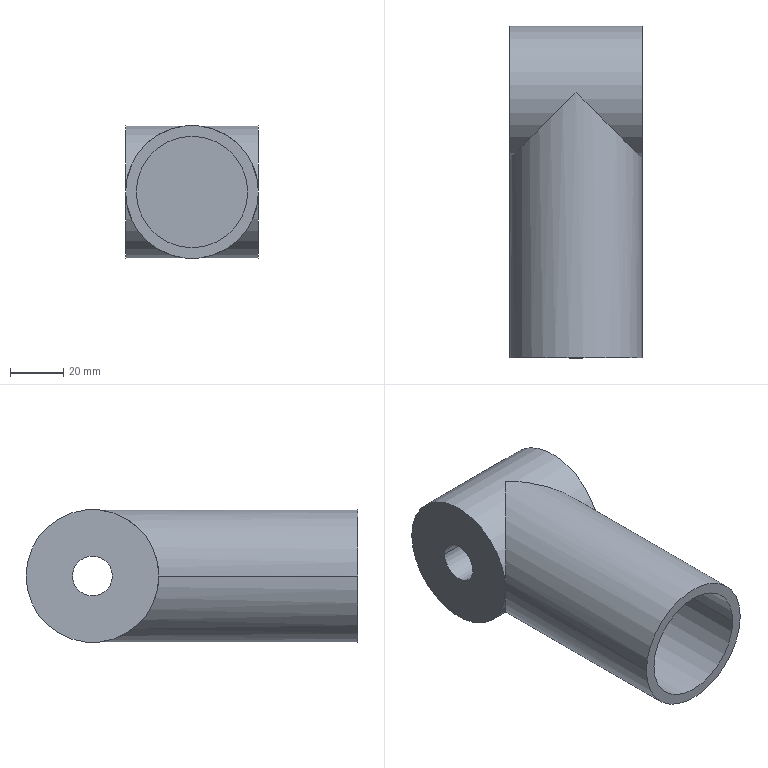Component | SolidWorks | CylinderHousing-2 | 2 solids | 14 faces | box 50 x 125 x 50 mm | volume 147041 mm3 | cylinder 10 | plane 4 | commonest cylinder face diameters 50 x6 42 x2 15 x2
build123d program:
from build123d import *

# Parameters (mm, degrees)
SKETCH1_R                            = 25
SKETCH1_R_2                          = 7.5
BOSS_EXTRUDE1_DEPTH                  = 50
SKETCH3_R                            = 25
BOSS_EXTRUDE2_DEPTH                  = 75
BOSS_EXTRUDE2_DIRECTION_2_REACH      = 334.603
BOSS_EXTRUDE2_DIRECTION_2_END_RADIUS = 25
SKETCH4_R                            = 21
CUT_EXTRUDE1_DEPTH                   = 70


with BuildPart() as part:
    # Sketch1 → Boss-Extrude1 (new body)
    with BuildSketch(Plane.XY):
        with Locations((-135, 300)):
            Circle(SKETCH1_R)
        with Locations((-135, 300)):
            Circle(SKETCH1_R_2, mode=Mode.SUBTRACT)
    extrude(amount=BOSS_EXTRUDE1_DEPTH)


with BuildPart() as body_2:
    # Sketch3 → Boss-Extrude2 (new body)
    with BuildSketch(Plane.ZY.offset(160)):
        with Locations(Location((25, 300, 0), (0, 0, 270))):
            Circle(SKETCH3_R)
    extrude(amount=BOSS_EXTRUDE2_DEPTH)

    # Boss-Extrude2 direction 2: up to this cylinder (the profile starts outside it)
    boss_extrude2_direction_2_end = Plane(origin=(-135, 300, 25), z_dir=(0, 0, -1)) * Cylinder(BOSS_EXTRUDE2_DIRECTION_2_END_RADIUS, 720.206, mode=Mode.PRIVATE)
    # Sketch3 → Boss-Extrude2 direction 2 (add, up to the surface)
    with BuildSketch(Plane.ZY.offset(160), mode=Mode.PRIVATE) as boss_extrude2_direction_2_sk1:
        with Locations(Location((25, 300, 0), (0, 0, 270))):
            Circle(SKETCH3_R)
    boss_extrude2_direction_2_tool1 = extrude(boss_extrude2_direction_2_sk1.sketch, amount=-BOSS_EXTRUDE2_DIRECTION_2_REACH, mode=Mode.PRIVATE) - boss_extrude2_direction_2_end
    add(boss_extrude2_direction_2_tool1.solids().sort_by_distance((-160, 300, 25))[0])
    add(boss_extrude2_direction_2_tool1.solids().sort_by_distance((-160, 300, 25))[1])

    # Sketch4 → Cut-Extrude1 (cut)
    with BuildSketch(Plane.ZY.offset(235)):
        with Locations((25, 300)):
            Circle(SKETCH4_R)
    extrude(amount=-CUT_EXTRUDE1_DEPTH, mode=Mode.SUBTRACT)


solid = Compound([part.part, body_2.part])

# Placed as in the assembly
solid = solid.moved(Location((-250, -100, -600), (90, 90, 0)))
STEP:
#1=COLOUR_RGB('',0.7922,0.8196,0.9333);
#2=FILL_AREA_STYLE_COLOUR('',#1);
#3=FILL_AREA_STYLE('',(#2));
#4=SURFACE_STYLE_FILL_AREA(#3);
#5=SURFACE_SIDE_STYLE('',(#4));
#6=SURFACE_STYLE_USAGE(.BOTH.,#5);
#7=PRESENTATION_STYLE_ASSIGNMENT((#6));
#8=CARTESIAN_POINT('',(-9.843,-9.547,-11.811));
#9=VERTEX_POINT('',#8);
#10=CARTESIAN_POINT('',(-9.843,-8.957,-11.811));
#11=VERTEX_POINT('',#10);
#12=CARTESIAN_POINT('',(-9.843,-9.252,-11.811));
#13=DIRECTION('',(-1.,0.,0.));
#14=DIRECTION('',(0.,1.,0.));
#15=AXIS2_PLACEMENT_3D('',#12,#13,#14);
#16=CIRCLE('',#15,0.2953);
#17=EDGE_CURVE('',#9,#11,#16,.T.);
#18=ORIENTED_EDGE('',*,*,#17,.T.);
#19=CARTESIAN_POINT('',(-7.874,-8.957,-11.811));
#20=VERTEX_POINT('',#19);
#21=CARTESIAN_POINT('',(-9.843,-8.957,-11.811));
#22=DIRECTION('',(1.,-0.,-0.));
#23=VECTOR('',#22,39.37);
#24=LINE('',#21,#23);
#25=EDGE_CURVE('',#11,#20,#24,.T.);
#26=ORIENTED_EDGE('',*,*,#25,.T.);
#27=CARTESIAN_POINT('',(-7.874,-9.547,-11.811));
#28=VERTEX_POINT('',#27);
#29=CARTESIAN_POINT('',(-7.874,-9.252,-11.811));
#30=DIRECTION('',(-1.,0.,0.));
#31=DIRECTION('',(0.,1.,0.));
#32=AXIS2_PLACEMENT_3D('',#29,#30,#31);
#33=CIRCLE('',#32,0.2953);
#34=EDGE_CURVE('',#28,#20,#33,.T.);
#35=ORIENTED_EDGE('',*,*,#34,.F.);
#36=CARTESIAN_POINT('',(-9.843,-9.547,-11.811));
#37=DIRECTION('',(1.,-0.,-0.));
#38=VECTOR('',#37,39.37);
#39=LINE('',#36,#38);
#40=EDGE_CURVE('',#9,#28,#39,.T.);
#41=ORIENTED_EDGE('',*,*,#40,.F.);
#42=EDGE_LOOP('',(#18,#26,#35,#41));
#43=FACE_OUTER_BOUND('',#42,.T.);
#44=CARTESIAN_POINT('',(-9.843,-9.252,-11.811));
#45=DIRECTION('',(1.,-0.,-0.));
#46=DIRECTION('',(0.,-1.,0.));
#47=AXIS2_PLACEMENT_3D('',#44,#45,#46);
#48=CYLINDRICAL_SURFACE('',#47,0.2953);
#49=ADVANCED_FACE('',(#43),#48,.F.);
#50=CARTESIAN_POINT('',(-9.843,-8.268,-11.811));
#51=VERTEX_POINT('',#50);
#52=CARTESIAN_POINT('',(-9.843,-10.236,-11.811));
#53=VERTEX_POINT('',#52);
#54=CARTESIAN_POINT('',(-9.843,-9.252,-11.811));
#55=DIRECTION('',(-1.,0.,0.));
#56=DIRECTION('',(0.,1.,0.));
#57=AXIS2_PLACEMENT_3D('',#54,#55,#56);
#58=CIRCLE('',#57,0.9843);
#59=EDGE_CURVE('',#51,#53,#58,.T.);
#60=ORIENTED_EDGE('',*,*,#59,.F.);
#61=CARTESIAN_POINT('',(-7.874,-8.268,-11.811));
#62=VERTEX_POINT('',#61);
#63=CARTESIAN_POINT('',(-9.843,-8.268,-11.811));
#64=DIRECTION('',(1.,-0.,-0.));
#65=VECTOR('',#64,39.37);
#66=LINE('',#63,#65);
#67=EDGE_CURVE('',#51,#62,#66,.T.);
#68=ORIENTED_EDGE('',*,*,#67,.T.);
#69=CARTESIAN_POINT('',(-7.874,-10.236,-11.811));
#70=VERTEX_POINT('',#69);
#71=CARTESIAN_POINT('',(-7.874,-9.252,-11.811));
#72=DIRECTION('',(-1.,0.,0.));
#73=DIRECTION('',(0.,1.,0.));
#74=AXIS2_PLACEMENT_3D('',#71,#72,#73);
#75=CIRCLE('',#74,0.9843);
#76=EDGE_CURVE('',#62,#70,#75,.T.);
#77=ORIENTED_EDGE('',*,*,#76,.T.);
#78=CARTESIAN_POINT('',(-9.843,-10.236,-11.811));
#79=DIRECTION('',(1.,-0.,-0.));
#80=VECTOR('',#79,39.37);
#81=LINE('',#78,#80);
#82=EDGE_CURVE('',#53,#70,#81,.T.);
#83=ORIENTED_EDGE('',*,*,#82,.F.);
#84=EDGE_LOOP('',(#60,#68,#77,#83));
#85=FACE_OUTER_BOUND('',#84,.T.);
#86=CARTESIAN_POINT('',(-9.843,-9.252,-11.811));
#87=DIRECTION('',(1.,-0.,-0.));
#88=DIRECTION('',(0.,-1.,0.));
#89=AXIS2_PLACEMENT_3D('',#86,#87,#88);
#90=CYLINDRICAL_SURFACE('',#89,0.9843);
#91=ADVANCED_FACE('',(#85),#90,.T.);
#92=CARTESIAN_POINT('',(-9.843,-9.252,-11.811));
#93=DIRECTION('',(-1.,0.,0.));
#94=DIRECTION('',(0.,1.,0.));
#95=AXIS2_PLACEMENT_3D('',#92,#93,#94);
#96=CIRCLE('',#95,0.9843);
#97=EDGE_CURVE('',#53,#51,#96,.T.);
#98=ORIENTED_EDGE('',*,*,#97,.T.);
#99=ORIENTED_EDGE('',*,*,#59,.T.);
#100=EDGE_LOOP('',(#98,#99));
#101=FACE_OUTER_BOUND('',#100,.T.);
#102=ORIENTED_EDGE('',*,*,#17,.F.);
#103=CARTESIAN_POINT('',(-9.843,-9.252,-11.811));
#104=DIRECTION('',(-1.,0.,0.));
#105=DIRECTION('',(0.,1.,0.));
#106=AXIS2_PLACEMENT_3D('',#103,#104,#105);
#107=CIRCLE('',#106,0.2953);
#108=EDGE_CURVE('',#11,#9,#107,.T.);
#109=ORIENTED_EDGE('',*,*,#108,.F.);
#110=EDGE_LOOP('',(#102,#109));
#111=FACE_BOUND('',#110,.T.);
#112=CARTESIAN_POINT('',(-9.843,-9.252,-11.811));
#113=DIRECTION('',(-1.,0.,0.));
#114=DIRECTION('',(0.,1.,0.));
#115=AXIS2_PLACEMENT_3D('',#112,#113,#114);
#116=PLANE('',#115);
#117=ADVANCED_FACE('',(#101,#111),#116,.T.);
#118=CARTESIAN_POINT('',(-7.874,-9.252,-11.811));
#119=DIRECTION('',(-1.,0.,0.));
#120=DIRECTION('',(0.,1.,0.));
#121=AXIS2_PLACEMENT_3D('',#118,#119,#120);
#122=CIRCLE('',#121,0.9843);
#123=EDGE_CURVE('',#70,#62,#122,.T.);
#124=ORIENTED_EDGE('',*,*,#123,.F.);
#125=ORIENTED_EDGE('',*,*,#76,.F.);
#126=EDGE_LOOP('',(#124,#125));
#127=FACE_OUTER_BOUND('',#126,.T.);
#128=ORIENTED_EDGE('',*,*,#34,.T.);
#129=CARTESIAN_POINT('',(-7.874,-9.252,-11.811));
#130=DIRECTION('',(-1.,0.,0.));
#131=DIRECTION('',(0.,1.,0.));
#132=AXIS2_PLACEMENT_3D('',#129,#130,#131);
#133=CIRCLE('',#132,0.2953);
#134=EDGE_CURVE('',#20,#28,#133,.T.);
#135=ORIENTED_EDGE('',*,*,#134,.T.);
#136=EDGE_LOOP('',(#128,#135));
#137=FACE_BOUND('',#136,.T.);
#138=CARTESIAN_POINT('',(-7.874,-9.252,-11.811));
#139=DIRECTION('',(-1.,0.,0.));
#140=DIRECTION('',(0.,1.,0.));
#141=AXIS2_PLACEMENT_3D('',#138,#139,#140);
#142=PLANE('',#141);
#143=ADVANCED_FACE('',(#127,#137),#142,.F.);
#144=ORIENTED_EDGE('',*,*,#67,.F.);
#145=ORIENTED_EDGE('',*,*,#97,.F.);
#146=ORIENTED_EDGE('',*,*,#82,.T.);
#147=ORIENTED_EDGE('',*,*,#123,.T.);
#148=EDGE_LOOP('',(#144,#145,#146,#147));
#149=FACE_OUTER_BOUND('',#148,.T.);
#150=CARTESIAN_POINT('',(-9.843,-9.252,-11.811));
#151=DIRECTION('',(1.,-0.,-0.));
#152=DIRECTION('',(0.,-1.,0.));
#153=AXIS2_PLACEMENT_3D('',#150,#151,#152);
#154=CYLINDRICAL_SURFACE('',#153,0.9843);
#155=ADVANCED_FACE('',(#149),#154,.T.);
#156=ORIENTED_EDGE('',*,*,#25,.F.);
#157=ORIENTED_EDGE('',*,*,#108,.T.);
#158=ORIENTED_EDGE('',*,*,#40,.T.);
#159=ORIENTED_EDGE('',*,*,#134,.F.);
#160=EDGE_LOOP('',(#156,#157,#158,#159));
#161=FACE_OUTER_BOUND('',#160,.T.);
#162=CARTESIAN_POINT('',(-9.843,-9.252,-11.811));
#163=DIRECTION('',(1.,-0.,-0.));
#164=DIRECTION('',(0.,-1.,0.));
#165=AXIS2_PLACEMENT_3D('',#162,#163,#164);
#166=CYLINDRICAL_SURFACE('',#165,0.2953);
#167=ADVANCED_FACE('',(#161),#166,.F.);
#168=CLOSED_SHELL('',(#49,#91,#117,#143,#155,#167));
#169=MANIFOLD_SOLID_BREP('',#168);
#170=STYLED_ITEM('',(#7),#169);
#171=PRESENTATION_LAYER_ASSIGNMENT('','',(#170));
#172=COLOUR_RGB('',0.7922,0.8196,0.9333);
#173=FILL_AREA_STYLE_COLOUR('',#172);
#174=FILL_AREA_STYLE('',(#173));
#175=SURFACE_STYLE_FILL_AREA(#174);
#176=SURFACE_SIDE_STYLE('',(#175));
#177=SURFACE_STYLE_USAGE(.BOTH.,#176);
#178=PRESENTATION_STYLE_ASSIGNMENT((#177));
#179=CARTESIAN_POINT('',(-8.031,-10.433,-11.811));
#180=VERTEX_POINT('',#179);
#181=CARTESIAN_POINT('',(-9.685,-10.433,-11.811));
#182=VERTEX_POINT('',#181);
#183=CARTESIAN_POINT('',(-8.858,-10.433,-11.811));
#184=DIRECTION('',(-0.,-1.,-0.));
#185=DIRECTION('',(-1.,0.,0.));
#186=AXIS2_PLACEMENT_3D('',#183,#184,#185);
#187=CIRCLE('',#186,0.8268);
#188=EDGE_CURVE('',#180,#182,#187,.T.);
#189=ORIENTED_EDGE('',*,*,#188,.F.);
#190=CARTESIAN_POINT('',(-8.031,-13.189,-11.811));
#191=VERTEX_POINT('',#190);
#192=CARTESIAN_POINT('',(-8.031,-10.433,-11.811));
#193=DIRECTION('',(-0.,-1.,-0.));
#194=VECTOR('',#193,39.37);
#195=LINE('',#192,#194);
#196=EDGE_CURVE('',#180,#191,#195,.T.);
#197=ORIENTED_EDGE('',*,*,#196,.T.);
#198=CARTESIAN_POINT('',(-9.685,-13.189,-11.811));
#199=VERTEX_POINT('',#198);
#200=CARTESIAN_POINT('',(-8.858,-13.189,-11.811));
#201=DIRECTION('',(-0.,-1.,-0.));
#202=DIRECTION('',(-1.,0.,0.));
#203=AXIS2_PLACEMENT_3D('',#200,#201,#202);
#204=CIRCLE('',#203,0.8268);
#205=EDGE_CURVE('',#191,#199,#204,.T.);
#206=ORIENTED_EDGE('',*,*,#205,.T.);
#207=CARTESIAN_POINT('',(-9.685,-10.433,-11.811));
#208=DIRECTION('',(-0.,-1.,-0.));
#209=VECTOR('',#208,39.37);
#210=LINE('',#207,#209);
#211=EDGE_CURVE('',#182,#199,#210,.T.);
#212=ORIENTED_EDGE('',*,*,#211,.F.);
#213=EDGE_LOOP('',(#189,#197,#206,#212));
#214=FACE_OUTER_BOUND('',#213,.T.);
#215=CARTESIAN_POINT('',(-8.858,-10.433,-11.811));
#216=DIRECTION('',(-0.,-1.,-0.));
#217=DIRECTION('',(-1.,0.,0.));
#218=AXIS2_PLACEMENT_3D('',#215,#216,#217);
#219=CYLINDRICAL_SURFACE('',#218,0.8268);
#220=ADVANCED_FACE('',(#214),#219,.F.);
#221=CARTESIAN_POINT('',(-9.843,-10.236,-11.811));
#222=VERTEX_POINT('',#221);
#223=CARTESIAN_POINT('',(-8.858,-9.252,-12.795));
#224=VERTEX_POINT('',#223);
#225=CARTESIAN_POINT('',(-9.843,-10.236,-11.811));
#226=CARTESIAN_POINT('',(-9.843,-10.236,-12.388));
#227=CARTESIAN_POINT('',(-9.435,-9.829,-12.795));
#228=CARTESIAN_POINT('',(-8.858,-9.252,-12.795));
#229=(BOUNDED_CURVE()B_SPLINE_CURVE(3,(#225,#226,#227,#228),.UNSPECIFIED.,.F.,.T.)B_SPLINE_CURVE_WITH_KNOTS((4,4),(-0.,1.571),.UNSPECIFIED.)CURVE()GEOMETRIC_REPRESENTATION_ITEM()RATIONAL_B_SPLINE_CURVE((1.,0.8047,0.8047,1.))REPRESENTATION_ITEM(''));
#230=EDGE_CURVE('',#222,#224,#229,.T.);
#231=ORIENTED_EDGE('',*,*,#230,.F.);
#232=CARTESIAN_POINT('',(-7.874,-10.236,-11.811));
#233=VERTEX_POINT('',#232);
#234=CARTESIAN_POINT('',(-9.843,-10.236,-11.811));
#235=DIRECTION('',(1.,-0.,-0.));
#236=VECTOR('',#235,39.37);
#237=LINE('',#234,#236);
#238=EDGE_CURVE('',#222,#233,#237,.T.);
#239=ORIENTED_EDGE('',*,*,#238,.T.);
#240=CARTESIAN_POINT('',(-8.858,-9.252,-12.795));
#241=CARTESIAN_POINT('',(-8.282,-9.829,-12.795));
#242=CARTESIAN_POINT('',(-7.874,-10.236,-12.388));
#243=CARTESIAN_POINT('',(-7.874,-10.236,-11.811));
#244=(BOUNDED_CURVE()B_SPLINE_CURVE(3,(#240,#241,#242,#243),.UNSPECIFIED.,.F.,.F.)B_SPLINE_CURVE_WITH_KNOTS((4,4),(4.712,6.283),.UNSPECIFIED.)CURVE()GEOMETRIC_REPRESENTATION_ITEM()RATIONAL_B_SPLINE_CURVE((1.,0.8047,0.8047,1.))REPRESENTATION_ITEM(''));
#245=EDGE_CURVE('',#224,#233,#244,.T.);
#246=ORIENTED_EDGE('',*,*,#245,.F.);
#247=EDGE_LOOP('',(#231,#239,#246));
#248=FACE_OUTER_BOUND('',#247,.T.);
#249=CARTESIAN_POINT('',(-9.843,-9.252,-11.811));
#250=DIRECTION('',(1.,-0.,-0.));
#251=DIRECTION('',(0.,-1.,0.));
#252=AXIS2_PLACEMENT_3D('',#249,#250,#251);
#253=CYLINDRICAL_SURFACE('',#252,0.9843);
#254=ADVANCED_FACE('',(#248),#253,.F.);
#255=CARTESIAN_POINT('',(-9.843,-13.189,-11.811));
#256=VERTEX_POINT('',#255);
#257=CARTESIAN_POINT('',(-7.874,-13.189,-11.811));
#258=VERTEX_POINT('',#257);
#259=CARTESIAN_POINT('',(-8.858,-13.189,-11.811));
#260=DIRECTION('',(-0.,-1.,-0.));
#261=DIRECTION('',(-1.,0.,0.));
#262=AXIS2_PLACEMENT_3D('',#259,#260,#261);
#263=CIRCLE('',#262,0.9843);
#264=EDGE_CURVE('',#256,#258,#263,.T.);
#265=ORIENTED_EDGE('',*,*,#264,.F.);
#266=CARTESIAN_POINT('',(-9.843,-13.189,-11.811));
#267=DIRECTION('',(0.,1.,0.));
#268=VECTOR('',#267,39.37);
#269=LINE('',#266,#268);
#270=EDGE_CURVE('',#256,#222,#269,.T.);
#271=ORIENTED_EDGE('',*,*,#270,.T.);
#272=ORIENTED_EDGE('',*,*,#230,.T.);
#273=ORIENTED_EDGE('',*,*,#245,.T.);
#274=CARTESIAN_POINT('',(-7.874,-13.189,-11.811));
#275=DIRECTION('',(0.,1.,0.));
#276=VECTOR('',#275,39.37);
#277=LINE('',#274,#276);
#278=EDGE_CURVE('',#258,#233,#277,.T.);
#279=ORIENTED_EDGE('',*,*,#278,.F.);
#280=EDGE_LOOP('',(#265,#271,#272,#273,#279));
#281=FACE_OUTER_BOUND('',#280,.T.);
#282=CARTESIAN_POINT('',(-8.858,-13.189,-11.811));
#283=DIRECTION('',(0.,1.,0.));
#284=DIRECTION('',(1.,0.,0.));
#285=AXIS2_PLACEMENT_3D('',#282,#283,#284);
#286=CYLINDRICAL_SURFACE('',#285,0.9843);
#287=ADVANCED_FACE('',(#281),#286,.T.);
#288=ORIENTED_EDGE('',*,*,#270,.F.);
#289=CARTESIAN_POINT('',(-8.858,-13.189,-11.811));
#290=DIRECTION('',(-0.,-1.,-0.));
#291=DIRECTION('',(-1.,0.,0.));
#292=AXIS2_PLACEMENT_3D('',#289,#290,#291);
#293=CIRCLE('',#292,0.9843);
#294=EDGE_CURVE('',#258,#256,#293,.T.);
#295=ORIENTED_EDGE('',*,*,#294,.F.);
#296=ORIENTED_EDGE('',*,*,#278,.T.);
#297=CARTESIAN_POINT('',(-8.858,-9.252,-10.827));
#298=VERTEX_POINT('',#297);
#299=CARTESIAN_POINT('',(-7.874,-10.236,-11.811));
#300=CARTESIAN_POINT('',(-7.874,-10.236,-11.234));
#301=CARTESIAN_POINT('',(-8.282,-9.829,-10.827));
#302=CARTESIAN_POINT('',(-8.858,-9.252,-10.827));
#303=(BOUNDED_CURVE()B_SPLINE_CURVE(3,(#299,#300,#301,#302),.UNSPECIFIED.,.F.,.T.)B_SPLINE_CURVE_WITH_KNOTS((4,4),(0.,1.571),.UNSPECIFIED.)CURVE()GEOMETRIC_REPRESENTATION_ITEM()RATIONAL_B_SPLINE_CURVE((1.,0.8047,0.8047,1.))REPRESENTATION_ITEM(''));
#304=EDGE_CURVE('',#233,#298,#303,.T.);
#305=ORIENTED_EDGE('',*,*,#304,.T.);
#306=CARTESIAN_POINT('',(-8.858,-9.252,-10.827));
#307=CARTESIAN_POINT('',(-9.435,-9.829,-10.827));
#308=CARTESIAN_POINT('',(-9.843,-10.236,-11.234));
#309=CARTESIAN_POINT('',(-9.843,-10.236,-11.811));
#310=(BOUNDED_CURVE()B_SPLINE_CURVE(3,(#306,#307,#308,#309),.UNSPECIFIED.,.F.,.T.)B_SPLINE_CURVE_WITH_KNOTS((4,4),(4.712,6.283),.UNSPECIFIED.)CURVE()GEOMETRIC_REPRESENTATION_ITEM()RATIONAL_B_SPLINE_CURVE((1.,0.8047,0.8047,1.))REPRESENTATION_ITEM(''));
#311=EDGE_CURVE('',#298,#222,#310,.T.);
#312=ORIENTED_EDGE('',*,*,#311,.T.);
#313=EDGE_LOOP('',(#288,#295,#296,#305,#312));
#314=FACE_OUTER_BOUND('',#313,.T.);
#315=CARTESIAN_POINT('',(-8.858,-13.189,-11.811));
#316=DIRECTION('',(0.,1.,0.));
#317=DIRECTION('',(1.,0.,0.));
#318=AXIS2_PLACEMENT_3D('',#315,#316,#317);
#319=CYLINDRICAL_SURFACE('',#318,0.9843);
#320=ADVANCED_FACE('',(#314),#319,.T.);
#321=CARTESIAN_POINT('',(-8.858,-13.189,-11.811));
#322=DIRECTION('',(-0.,-1.,-0.));
#323=DIRECTION('',(-1.,0.,0.));
#324=AXIS2_PLACEMENT_3D('',#321,#322,#323);
#325=CIRCLE('',#324,0.8268);
#326=EDGE_CURVE('',#199,#191,#325,.T.);
#327=ORIENTED_EDGE('',*,*,#326,.F.);
#328=ORIENTED_EDGE('',*,*,#205,.F.);
#329=EDGE_LOOP('',(#327,#328));
#330=FACE_BOUND('',#329,.T.);
#331=ORIENTED_EDGE('',*,*,#294,.T.);
#332=ORIENTED_EDGE('',*,*,#264,.T.);
#333=EDGE_LOOP('',(#331,#332));
#334=FACE_OUTER_BOUND('',#333,.T.);
#335=CARTESIAN_POINT('',(-8.858,-13.189,-11.811));
#336=DIRECTION('',(-0.,-1.,-0.));
#337=DIRECTION('',(-1.,0.,0.));
#338=AXIS2_PLACEMENT_3D('',#335,#336,#337);
#339=PLANE('',#338);
#340=ADVANCED_FACE('',(#330,#334),#339,.T.);
#341=ORIENTED_EDGE('',*,*,#238,.F.);
#342=ORIENTED_EDGE('',*,*,#311,.F.);
#343=ORIENTED_EDGE('',*,*,#304,.F.);
#344=EDGE_LOOP('',(#341,#342,#343));
#345=FACE_OUTER_BOUND('',#344,.T.);
#346=CARTESIAN_POINT('',(-9.843,-9.252,-11.811));
#347=DIRECTION('',(1.,-0.,-0.));
#348=DIRECTION('',(0.,-1.,0.));
#349=AXIS2_PLACEMENT_3D('',#346,#347,#348);
#350=CYLINDRICAL_SURFACE('',#349,0.9843);
#351=ADVANCED_FACE('',(#345),#350,.F.);
#352=ORIENTED_EDGE('',*,*,#196,.F.);
#353=CARTESIAN_POINT('',(-8.858,-10.433,-11.811));
#354=DIRECTION('',(-0.,-1.,-0.));
#355=DIRECTION('',(-1.,0.,0.));
#356=AXIS2_PLACEMENT_3D('',#353,#354,#355);
#357=CIRCLE('',#356,0.8268);
#358=EDGE_CURVE('',#182,#180,#357,.T.);
#359=ORIENTED_EDGE('',*,*,#358,.F.);
#360=ORIENTED_EDGE('',*,*,#211,.T.);
#361=ORIENTED_EDGE('',*,*,#326,.T.);
#362=EDGE_LOOP('',(#352,#359,#360,#361));
#363=FACE_OUTER_BOUND('',#362,.T.);
#364=CARTESIAN_POINT('',(-8.858,-10.433,-11.811));
#365=DIRECTION('',(-0.,-1.,-0.));
#366=DIRECTION('',(-1.,0.,0.));
#367=AXIS2_PLACEMENT_3D('',#364,#365,#366);
#368=CYLINDRICAL_SURFACE('',#367,0.8268);
#369=ADVANCED_FACE('',(#363),#368,.F.);
#370=ORIENTED_EDGE('',*,*,#358,.T.);
#371=ORIENTED_EDGE('',*,*,#188,.T.);
#372=EDGE_LOOP('',(#370,#371));
#373=FACE_OUTER_BOUND('',#372,.T.);
#374=CARTESIAN_POINT('',(-8.858,-10.433,-11.811));
#375=DIRECTION('',(-0.,-1.,-0.));
#376=DIRECTION('',(-1.,0.,0.));
#377=AXIS2_PLACEMENT_3D('',#374,#375,#376);
#378=PLANE('',#377);
#379=ADVANCED_FACE('',(#373),#378,.T.);
#380=CLOSED_SHELL('',(#220,#254,#287,#320,#340,#351,#369,#379));
#381=MANIFOLD_SOLID_BREP('',#380);
#382=STYLED_ITEM('',(#178),#381);
#383=PRESENTATION_LAYER_ASSIGNMENT('','',(#382));
#384=CARTESIAN_POINT('',(0.,0.,0.));
#385=DIRECTION('',(0.,0.,1.));
#386=DIRECTION('',(1.,0.,0.));
#387=AXIS2_PLACEMENT_3D('',#384,#385,#386);
#388=(LENGTH_UNIT()NAMED_UNIT(*)SI_UNIT($,.METRE.));
#389=LENGTH_MEASURE_WITH_UNIT(LENGTH_MEASURE(0.0254),#388);
#390=DIMENSIONAL_EXPONENTS(1.,0.,0.,0.,0.,0.,0.);
#391=(CONVERSION_BASED_UNIT('',#389)LENGTH_UNIT()NAMED_UNIT(#390));
#392=UNCERTAINTY_MEASURE_WITH_UNIT(LENGTH_MEASURE(0.00001),#391,'','');
#393=(NAMED_UNIT(*)PLANE_ANGLE_UNIT()SI_UNIT($,.RADIAN.));
#394=(NAMED_UNIT(*)SI_UNIT($,.STERADIAN.)SOLID_ANGLE_UNIT());
#395=(GEOMETRIC_REPRESENTATION_CONTEXT(3)GLOBAL_UNCERTAINTY_ASSIGNED_CONTEXT((#392))GLOBAL_UNIT_ASSIGNED_CONTEXT((#391,#393,#394))REPRESENTATION_CONTEXT('',''));
#396=ADVANCED_BREP_SHAPE_REPRESENTATION('',(#381,#169,#387),#395);
#397=(LENGTH_UNIT()NAMED_UNIT(*)SI_UNIT($,.METRE.));
#398=LENGTH_MEASURE_WITH_UNIT(LENGTH_MEASURE(0.0254),#397);
#399=DIMENSIONAL_EXPONENTS(1.,0.,0.,0.,0.,0.,0.);
#400=(CONVERSION_BASED_UNIT('',#398)LENGTH_UNIT()NAMED_UNIT(#399));
#401=UNCERTAINTY_MEASURE_WITH_UNIT(LENGTH_MEASURE(0.00001),#400,'','');
#402=(NAMED_UNIT(*)PLANE_ANGLE_UNIT()SI_UNIT($,.RADIAN.));
#403=(NAMED_UNIT(*)SI_UNIT($,.STERADIAN.)SOLID_ANGLE_UNIT());
#404=(GEOMETRIC_REPRESENTATION_CONTEXT(3)GLOBAL_UNCERTAINTY_ASSIGNED_CONTEXT((#401))GLOBAL_UNIT_ASSIGNED_CONTEXT((#400,#402,#403))REPRESENTATION_CONTEXT('',''));
#405=MECHANICAL_DESIGN_GEOMETRIC_PRESENTATION_REPRESENTATION('',(#382),#404);
#406=(LENGTH_UNIT()NAMED_UNIT(*)SI_UNIT($,.METRE.));
#407=LENGTH_MEASURE_WITH_UNIT(LENGTH_MEASURE(0.0254),#406);
#408=DIMENSIONAL_EXPONENTS(1.,0.,0.,0.,0.,0.,0.);
#409=(CONVERSION_BASED_UNIT('',#407)LENGTH_UNIT()NAMED_UNIT(#408));
#410=UNCERTAINTY_MEASURE_WITH_UNIT(LENGTH_MEASURE(0.00001),#409,'','');
#411=(NAMED_UNIT(*)PLANE_ANGLE_UNIT()SI_UNIT($,.RADIAN.));
#412=(NAMED_UNIT(*)SI_UNIT($,.STERADIAN.)SOLID_ANGLE_UNIT());
#413=(GEOMETRIC_REPRESENTATION_CONTEXT(3)GLOBAL_UNCERTAINTY_ASSIGNED_CONTEXT((#410))GLOBAL_UNIT_ASSIGNED_CONTEXT((#409,#411,#412))REPRESENTATION_CONTEXT('',''));
#414=MECHANICAL_DESIGN_GEOMETRIC_PRESENTATION_REPRESENTATION('',(#170),#413);